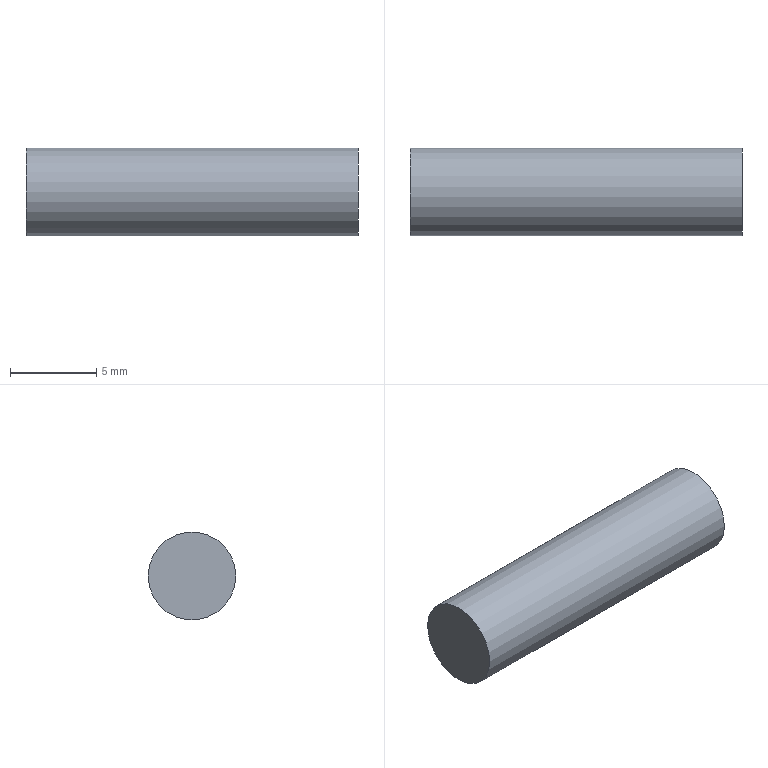Component | NX | PIN | 1 solid | 3 faces | box 19.3 x 5.1 x 5.1 mm | volume 394 mm3 | plane 2 | cylinder 1 | commonest cylinder face diameters 5.1 x1
STEP:
#1=CARTESIAN_POINT('',(0.,0.,0.));
#2=DIRECTION('',(0.,0.,1.));
#3=DIRECTION('',(1.,0.,0.));
#4=AXIS2_PLACEMENT_3D('',#1,#2,#3);
#5=CARTESIAN_POINT('',(16.872,94.052,4.75));
#6=VERTEX_POINT('',#5);
#7=CARTESIAN_POINT('',(16.872,91.502,4.75));
#8=DIRECTION('',(-1.,0.,0.));
#9=DIRECTION('',(0.,1.,0.));
#10=AXIS2_PLACEMENT_3D('',#7,#8,#9);
#11=CIRCLE('',#10,2.55);
#12=CARTESIAN_POINT('',(16.872,91.502,4.75));
#13=DIRECTION('',(1.,0.,0.));
#14=DIRECTION('',(0.,-1.,0.));
#15=AXIS2_PLACEMENT_3D('',#12,#13,#14);
#16=CYLINDRICAL_SURFACE('',#15,2.55);
#17=CARTESIAN_POINT('',(9.425,0.));
#18=DIRECTION('',(-1.,0.));
#19=VECTOR('',#18,1.);
#20=LINE('',#17,#19);
#21=(GEOMETRIC_REPRESENTATION_CONTEXT(2)PARAMETRIC_REPRESENTATION_CONTEXT()REPRESENTATION_CONTEXT('',''));
#22=DEFINITIONAL_REPRESENTATION('',(#20),#21);
#23=PCURVE('',#16,#22);
#24=CARTESIAN_POINT('',(16.872,91.502,4.75));
#25=DIRECTION('',(-1.,0.,0.));
#26=DIRECTION('',(0.,1.,0.));
#27=AXIS2_PLACEMENT_3D('',#24,#25,#26);
#28=PLANE('',#27);
#29=CARTESIAN_POINT('',(0.,0.));
#30=DIRECTION('',(1.,0.));
#31=AXIS2_PLACEMENT_2D('',#29,#30);
#32=CIRCLE('',#31,2.55);
#33=(GEOMETRIC_REPRESENTATION_CONTEXT(2)PARAMETRIC_REPRESENTATION_CONTEXT()REPRESENTATION_CONTEXT('',''));
#34=DEFINITIONAL_REPRESENTATION('',(#32),#33);
#35=PCURVE('',#28,#34);
#36=SURFACE_CURVE('',#11,(#23,#35),.PCURVE_S1.);
#37=EDGE_CURVE('',#6,#6,#36,.T.);
#38=ORIENTED_EDGE('',*,*,#37,.F.);
#39=CARTESIAN_POINT('',(36.172,94.052,4.75));
#40=VERTEX_POINT('',#39);
#41=CARTESIAN_POINT('',(16.872,94.052,4.75));
#42=CARTESIAN_POINT('',(36.172,94.052,4.75));
#43=B_SPLINE_CURVE_WITH_KNOTS('',1,(#41,#42),.UNSPECIFIED.,.F.,.F.,(2,2),(0.,19.3),.PIECEWISE_BEZIER_KNOTS.);
#44=CARTESIAN_POINT('',(9.425,0.));
#45=DIRECTION('',(0.,1.));
#46=VECTOR('',#45,1.);
#47=LINE('',#44,#46);
#48=(GEOMETRIC_REPRESENTATION_CONTEXT(2)PARAMETRIC_REPRESENTATION_CONTEXT()REPRESENTATION_CONTEXT('',''));
#49=DEFINITIONAL_REPRESENTATION('',(#47),#48);
#50=PCURVE('',#16,#49);
#51=CARTESIAN_POINT('',(3.142,0.));
#52=DIRECTION('',(0.,1.));
#53=VECTOR('',#52,1.);
#54=LINE('',#51,#53);
#55=(GEOMETRIC_REPRESENTATION_CONTEXT(2)PARAMETRIC_REPRESENTATION_CONTEXT()REPRESENTATION_CONTEXT('',''));
#56=DEFINITIONAL_REPRESENTATION('',(#54),#55);
#57=PCURVE('',#16,#56);
#58=SEAM_CURVE('',#43,(#50,#57),.PCURVE_S1.);
#59=EDGE_CURVE('',#6,#40,#58,.T.);
#60=ORIENTED_EDGE('',*,*,#59,.T.);
#61=CARTESIAN_POINT('',(36.172,91.502,4.75));
#62=DIRECTION('',(-1.,0.,0.));
#63=DIRECTION('',(0.,1.,0.));
#64=AXIS2_PLACEMENT_3D('',#61,#62,#63);
#65=CIRCLE('',#64,2.55);
#66=CARTESIAN_POINT('',(9.425,19.3));
#67=DIRECTION('',(-1.,0.));
#68=VECTOR('',#67,1.);
#69=LINE('',#66,#68);
#70=(GEOMETRIC_REPRESENTATION_CONTEXT(2)PARAMETRIC_REPRESENTATION_CONTEXT()REPRESENTATION_CONTEXT('',''));
#71=DEFINITIONAL_REPRESENTATION('',(#69),#70);
#72=PCURVE('',#16,#71);
#73=CARTESIAN_POINT('',(36.172,91.502,4.75));
#74=DIRECTION('',(-1.,0.,0.));
#75=DIRECTION('',(0.,1.,0.));
#76=AXIS2_PLACEMENT_3D('',#73,#74,#75);
#77=PLANE('',#76);
#78=CARTESIAN_POINT('',(0.,0.));
#79=DIRECTION('',(1.,0.));
#80=AXIS2_PLACEMENT_2D('',#78,#79);
#81=CIRCLE('',#80,2.55);
#82=(GEOMETRIC_REPRESENTATION_CONTEXT(2)PARAMETRIC_REPRESENTATION_CONTEXT()REPRESENTATION_CONTEXT('',''));
#83=DEFINITIONAL_REPRESENTATION('',(#81),#82);
#84=PCURVE('',#77,#83);
#85=SURFACE_CURVE('',#65,(#72,#84),.PCURVE_S1.);
#86=EDGE_CURVE('',#40,#40,#85,.T.);
#87=ORIENTED_EDGE('',*,*,#86,.T.);
#88=ORIENTED_EDGE('',*,*,#59,.F.);
#89=EDGE_LOOP('',(#38,#60,#87,#88));
#90=FACE_BOUND('',#89,.T.);
#91=ADVANCED_FACE('',(#90),#16,.T.);
#92=ORIENTED_EDGE('',*,*,#37,.T.);
#93=EDGE_LOOP('',(#92));
#94=FACE_BOUND('',#93,.T.);
#95=ADVANCED_FACE('',(#94),#28,.T.);
#96=ORIENTED_EDGE('',*,*,#86,.F.);
#97=EDGE_LOOP('',(#96));
#98=FACE_BOUND('',#97,.T.);
#99=ADVANCED_FACE('',(#98),#77,.F.);
#100=CLOSED_SHELL('',(#91,#95,#99));
#101=MANIFOLD_SOLID_BREP('',#100);
#102=(LENGTH_UNIT()NAMED_UNIT(*)SI_UNIT(.MILLI.,.METRE.));
#103=UNCERTAINTY_MEASURE_WITH_UNIT(LENGTH_MEASURE(0.00001),#102,'','');
#104=(NAMED_UNIT(*)PLANE_ANGLE_UNIT()SI_UNIT($,.RADIAN.));
#105=(NAMED_UNIT(*)SI_UNIT($,.STERADIAN.)SOLID_ANGLE_UNIT());
#106=(GEOMETRIC_REPRESENTATION_CONTEXT(3)GLOBAL_UNCERTAINTY_ASSIGNED_CONTEXT((#103))GLOBAL_UNIT_ASSIGNED_CONTEXT((#102,#104,#105))REPRESENTATION_CONTEXT('',''));
#107=ADVANCED_BREP_SHAPE_REPRESENTATION('',(#4,#101),#106);